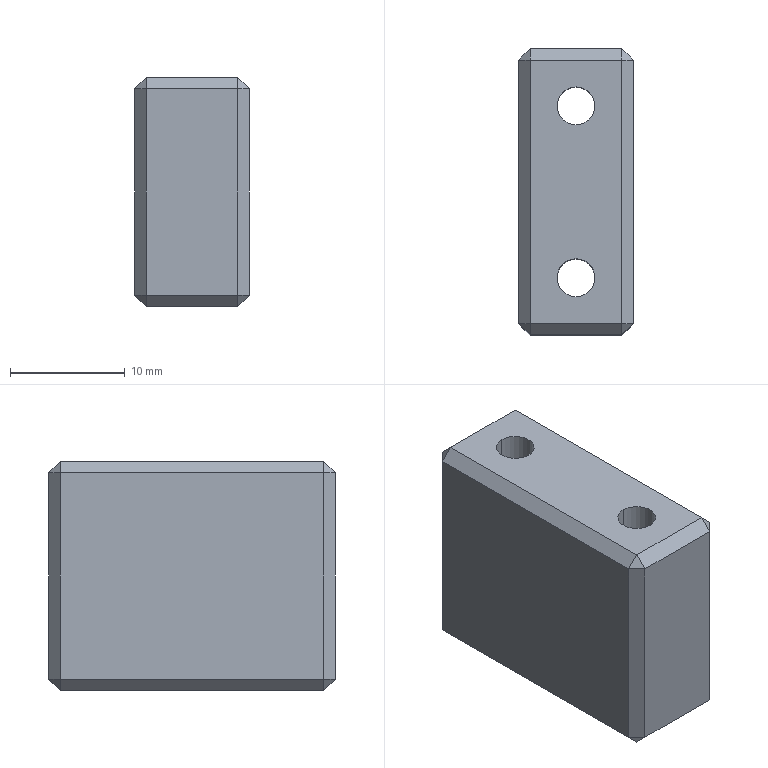Component | SolidWorks | SL010-RightStreamline-1-1_SL010-BeltMotorAssembly-1-1_SL010-LXFB-0102008-1-2 | 1 solid | 30 faces | box 10 x 25 x 20 mm | volume 4553 mm3 | plane 26 | cylinder 4 | commonest cylinder face diameters 3.3 x4 | material Aluminum-6061
build123d program:
from build123d import *

# Parameters (mm, degrees)
SKETCH1_W           = 10
SKETCH1_H           = 25
BOSS_EXTRUDE1_DEPTH = 10
M4_TAPPED_HOLE1_D   = 3.3
CHAMFER1_SIZE       = 1


with BuildPart() as part:
    # Sketch1 → Boss-Extrude1 (new, symmetric)
    with BuildSketch(Plane(origin=(0, 0, 0), x_dir=(1, 0, 0), z_dir=(0, 1, 0))):
        Rectangle(SKETCH1_W, SKETCH1_H)
    extrude(amount=BOSS_EXTRUDE1_DEPTH, both=True)

    # M4 Tapped Hole1 (through all)
    with Locations(Plane(origin=(0, 10, 0), x_dir=(1, 0, 0), z_dir=(0, 1, 0))):
        with Locations((0, -7.5), (0, 7.5)):
            Hole(M4_TAPPED_HOLE1_D / 2)

    # Chamfer1
    chamfer1_edges = [part.edges().sort_by_distance(p)[0] for p in [
        (5, 10, 0),
        (0, 10, -12.5),
        (-5, 10, 0),
        (0, -10, -12.5),
        (5, -10, 0),
        (0, -10, 12.5),
        (-5, -10, 0),
        (0, 10, 12.5),
        (-5, 0, -12.5),
        (5, 0, -12.5),
        (5, 0, 12.5),
        (-5, 0, 12.5),
    ]]
    chamfer(chamfer1_edges, length=CHAMFER1_SIZE)


solid = part.part

# Placed as in the assembly
solid = solid.moved(Location((-547.5, -215.404, -306.035), (90, 0, 0)))
STEP:
#1=COLOUR_RGB('',0.7922,0.8196,0.9333);
#2=FILL_AREA_STYLE_COLOUR('',#1);
#3=FILL_AREA_STYLE('',(#2));
#4=SURFACE_STYLE_FILL_AREA(#3);
#5=SURFACE_SIDE_STYLE('',(#4));
#6=SURFACE_STYLE_USAGE(.BOTH.,#5);
#7=PRESENTATION_STYLE_ASSIGNMENT((#6));
#8=CARTESIAN_POINT('',(-21.555,-8.25,-12.442));
#9=VERTEX_POINT('',#8);
#10=CARTESIAN_POINT('',(-21.555,-8.12,-12.442));
#11=VERTEX_POINT('',#10);
#12=CARTESIAN_POINT('',(-21.555,-8.185,-12.442));
#13=DIRECTION('',(0.,-0.,1.));
#14=DIRECTION('',(0.,1.,0.));
#15=AXIS2_PLACEMENT_3D('',#12,#13,#14);
#16=CIRCLE('',#15,0.06496);
#17=EDGE_CURVE('',#9,#11,#16,.T.);
#18=ORIENTED_EDGE('',*,*,#17,.F.);
#19=CARTESIAN_POINT('',(-21.555,-8.25,-11.655));
#20=VERTEX_POINT('',#19);
#21=CARTESIAN_POINT('',(-21.555,-8.25,-11.655));
#22=DIRECTION('',(0.,-0.,1.));
#23=VECTOR('',#22,39.37);
#24=LINE('',#21,#23);
#25=EDGE_CURVE('',#9,#20,#24,.T.);
#26=ORIENTED_EDGE('',*,*,#25,.T.);
#27=CARTESIAN_POINT('',(-21.555,-8.12,-11.655));
#28=VERTEX_POINT('',#27);
#29=CARTESIAN_POINT('',(-21.555,-8.185,-11.655));
#30=DIRECTION('',(0.,-0.,1.));
#31=DIRECTION('',(0.,1.,0.));
#32=AXIS2_PLACEMENT_3D('',#29,#30,#31);
#33=CIRCLE('',#32,0.06496);
#34=EDGE_CURVE('',#20,#28,#33,.T.);
#35=ORIENTED_EDGE('',*,*,#34,.T.);
#36=CARTESIAN_POINT('',(-21.555,-8.12,-11.655));
#37=DIRECTION('',(0.,-0.,1.));
#38=VECTOR('',#37,39.37);
#39=LINE('',#36,#38);
#40=EDGE_CURVE('',#11,#28,#39,.T.);
#41=ORIENTED_EDGE('',*,*,#40,.F.);
#42=EDGE_LOOP('',(#18,#26,#35,#41));
#43=FACE_OUTER_BOUND('',#42,.T.);
#44=CARTESIAN_POINT('',(-21.555,-8.185,-11.655));
#45=DIRECTION('',(0.,-0.,1.));
#46=DIRECTION('',(0.,1.,0.));
#47=AXIS2_PLACEMENT_3D('',#44,#45,#46);
#48=CYLINDRICAL_SURFACE('',#47,0.06496);
#49=ADVANCED_FACE('',(#43),#48,.F.);
#50=CARTESIAN_POINT('',(-21.555,-8.841,-12.442));
#51=VERTEX_POINT('',#50);
#52=CARTESIAN_POINT('',(-21.555,-8.711,-12.442));
#53=VERTEX_POINT('',#52);
#54=CARTESIAN_POINT('',(-21.555,-8.776,-12.442));
#55=DIRECTION('',(0.,-0.,1.));
#56=DIRECTION('',(0.,1.,0.));
#57=AXIS2_PLACEMENT_3D('',#54,#55,#56);
#58=CIRCLE('',#57,0.06496);
#59=EDGE_CURVE('',#51,#53,#58,.T.);
#60=ORIENTED_EDGE('',*,*,#59,.F.);
#61=CARTESIAN_POINT('',(-21.555,-8.841,-11.655));
#62=VERTEX_POINT('',#61);
#63=CARTESIAN_POINT('',(-21.555,-8.841,-11.655));
#64=DIRECTION('',(0.,-0.,1.));
#65=VECTOR('',#64,39.37);
#66=LINE('',#63,#65);
#67=EDGE_CURVE('',#51,#62,#66,.T.);
#68=ORIENTED_EDGE('',*,*,#67,.T.);
#69=CARTESIAN_POINT('',(-21.555,-8.711,-11.655));
#70=VERTEX_POINT('',#69);
#71=CARTESIAN_POINT('',(-21.555,-8.776,-11.655));
#72=DIRECTION('',(0.,-0.,1.));
#73=DIRECTION('',(0.,1.,0.));
#74=AXIS2_PLACEMENT_3D('',#71,#72,#73);
#75=CIRCLE('',#74,0.06496);
#76=EDGE_CURVE('',#62,#70,#75,.T.);
#77=ORIENTED_EDGE('',*,*,#76,.T.);
#78=CARTESIAN_POINT('',(-21.555,-8.711,-11.655));
#79=DIRECTION('',(0.,-0.,1.));
#80=VECTOR('',#79,39.37);
#81=LINE('',#78,#80);
#82=EDGE_CURVE('',#53,#70,#81,.T.);
#83=ORIENTED_EDGE('',*,*,#82,.F.);
#84=EDGE_LOOP('',(#60,#68,#77,#83));
#85=FACE_OUTER_BOUND('',#84,.T.);
#86=CARTESIAN_POINT('',(-21.555,-8.776,-11.655));
#87=DIRECTION('',(0.,-0.,1.));
#88=DIRECTION('',(0.,1.,0.));
#89=AXIS2_PLACEMENT_3D('',#86,#87,#88);
#90=CYLINDRICAL_SURFACE('',#89,0.06496);
#91=ADVANCED_FACE('',(#85),#90,.F.);
#92=CARTESIAN_POINT('',(-21.358,-8.028,-11.694));
#93=VERTEX_POINT('',#92);
#94=CARTESIAN_POINT('',(-21.358,-8.933,-11.694));
#95=VERTEX_POINT('',#94);
#96=CARTESIAN_POINT('',(-21.358,-8.973,-11.694));
#97=DIRECTION('',(-0.,-1.,-0.));
#98=VECTOR('',#97,39.37);
#99=LINE('',#96,#98);
#100=EDGE_CURVE('',#93,#95,#99,.T.);
#101=ORIENTED_EDGE('',*,*,#100,.T.);
#102=CARTESIAN_POINT('',(-21.358,-8.933,-12.403));
#103=VERTEX_POINT('',#102);
#104=CARTESIAN_POINT('',(-21.358,-8.933,-11.655));
#105=DIRECTION('',(0.,0.,-1.));
#106=VECTOR('',#105,39.37);
#107=LINE('',#104,#106);
#108=EDGE_CURVE('',#95,#103,#107,.T.);
#109=ORIENTED_EDGE('',*,*,#108,.T.);
#110=CARTESIAN_POINT('',(-21.358,-8.028,-12.403));
#111=VERTEX_POINT('',#110);
#112=CARTESIAN_POINT('',(-21.358,-7.988,-12.403));
#113=DIRECTION('',(0.,1.,0.));
#114=VECTOR('',#113,39.37);
#115=LINE('',#112,#114);
#116=EDGE_CURVE('',#103,#111,#115,.T.);
#117=ORIENTED_EDGE('',*,*,#116,.T.);
#118=CARTESIAN_POINT('',(-21.358,-8.028,-11.655));
#119=DIRECTION('',(0.,-0.,1.));
#120=VECTOR('',#119,39.37);
#121=LINE('',#118,#120);
#122=EDGE_CURVE('',#111,#93,#121,.T.);
#123=ORIENTED_EDGE('',*,*,#122,.T.);
#124=EDGE_LOOP('',(#101,#109,#117,#123));
#125=FACE_OUTER_BOUND('',#124,.T.);
#126=CARTESIAN_POINT('',(-21.358,-7.988,-11.655));
#127=DIRECTION('',(-1.,0.,-0.));
#128=DIRECTION('',(-0.,-1.,-0.));
#129=AXIS2_PLACEMENT_3D('',#126,#127,#128);
#130=PLANE('',#129);
#131=ADVANCED_FACE('',(#125),#130,.F.);
#132=CARTESIAN_POINT('',(-21.398,-7.988,-12.403));
#133=VERTEX_POINT('',#132);
#134=CARTESIAN_POINT('',(-21.713,-7.988,-12.403));
#135=VERTEX_POINT('',#134);
#136=CARTESIAN_POINT('',(-21.752,-7.988,-12.403));
#137=DIRECTION('',(-1.,-0.,-0.));
#138=VECTOR('',#137,39.37);
#139=LINE('',#136,#138);
#140=EDGE_CURVE('',#133,#135,#139,.T.);
#141=ORIENTED_EDGE('',*,*,#140,.T.);
#142=CARTESIAN_POINT('',(-21.713,-7.988,-11.694));
#143=VERTEX_POINT('',#142);
#144=CARTESIAN_POINT('',(-21.713,-7.988,-11.655));
#145=DIRECTION('',(0.,-0.,1.));
#146=VECTOR('',#145,39.37);
#147=LINE('',#144,#146);
#148=EDGE_CURVE('',#135,#143,#147,.T.);
#149=ORIENTED_EDGE('',*,*,#148,.T.);
#150=CARTESIAN_POINT('',(-21.398,-7.988,-11.694));
#151=VERTEX_POINT('',#150);
#152=CARTESIAN_POINT('',(-21.358,-7.988,-11.694));
#153=DIRECTION('',(1.,0.,0.));
#154=VECTOR('',#153,39.37);
#155=LINE('',#152,#154);
#156=EDGE_CURVE('',#143,#151,#155,.T.);
#157=ORIENTED_EDGE('',*,*,#156,.T.);
#158=CARTESIAN_POINT('',(-21.398,-7.988,-11.655));
#159=DIRECTION('',(0.,0.,-1.));
#160=VECTOR('',#159,39.37);
#161=LINE('',#158,#160);
#162=EDGE_CURVE('',#151,#133,#161,.T.);
#163=ORIENTED_EDGE('',*,*,#162,.T.);
#164=EDGE_LOOP('',(#141,#149,#157,#163));
#165=FACE_OUTER_BOUND('',#164,.T.);
#166=CARTESIAN_POINT('',(-21.752,-7.988,-11.655));
#167=DIRECTION('',(0.,-1.,-0.));
#168=DIRECTION('',(1.,0.,0.));
#169=AXIS2_PLACEMENT_3D('',#166,#167,#168);
#170=PLANE('',#169);
#171=ADVANCED_FACE('',(#165),#170,.F.);
#172=CARTESIAN_POINT('',(-21.752,-8.933,-11.694));
#173=VERTEX_POINT('',#172);
#174=CARTESIAN_POINT('',(-21.752,-8.028,-11.694));
#175=VERTEX_POINT('',#174);
#176=CARTESIAN_POINT('',(-21.752,-7.988,-11.694));
#177=DIRECTION('',(0.,1.,0.));
#178=VECTOR('',#177,39.37);
#179=LINE('',#176,#178);
#180=EDGE_CURVE('',#173,#175,#179,.T.);
#181=ORIENTED_EDGE('',*,*,#180,.T.);
#182=CARTESIAN_POINT('',(-21.752,-8.028,-12.403));
#183=VERTEX_POINT('',#182);
#184=CARTESIAN_POINT('',(-21.752,-8.028,-11.655));
#185=DIRECTION('',(0.,0.,-1.));
#186=VECTOR('',#185,39.37);
#187=LINE('',#184,#186);
#188=EDGE_CURVE('',#175,#183,#187,.T.);
#189=ORIENTED_EDGE('',*,*,#188,.T.);
#190=CARTESIAN_POINT('',(-21.752,-8.933,-12.403));
#191=VERTEX_POINT('',#190);
#192=CARTESIAN_POINT('',(-21.752,-7.988,-12.403));
#193=DIRECTION('',(-0.,-1.,-0.));
#194=VECTOR('',#193,39.37);
#195=LINE('',#192,#194);
#196=EDGE_CURVE('',#183,#191,#195,.T.);
#197=ORIENTED_EDGE('',*,*,#196,.T.);
#198=CARTESIAN_POINT('',(-21.752,-8.933,-11.655));
#199=DIRECTION('',(0.,-0.,1.));
#200=VECTOR('',#199,39.37);
#201=LINE('',#198,#200);
#202=EDGE_CURVE('',#191,#173,#201,.T.);
#203=ORIENTED_EDGE('',*,*,#202,.T.);
#204=EDGE_LOOP('',(#181,#189,#197,#203));
#205=FACE_OUTER_BOUND('',#204,.T.);
#206=CARTESIAN_POINT('',(-21.752,-7.988,-11.655));
#207=DIRECTION('',(1.,-0.,0.));
#208=DIRECTION('',(0.,1.,0.));
#209=AXIS2_PLACEMENT_3D('',#206,#207,#208);
#210=PLANE('',#209);
#211=ADVANCED_FACE('',(#205),#210,.F.);
#212=CARTESIAN_POINT('',(-21.398,-8.973,-12.403));
#213=VERTEX_POINT('',#212);
#214=CARTESIAN_POINT('',(-21.398,-8.973,-11.694));
#215=VERTEX_POINT('',#214);
#216=CARTESIAN_POINT('',(-21.398,-8.973,-11.655));
#217=DIRECTION('',(0.,-0.,1.));
#218=VECTOR('',#217,39.37);
#219=LINE('',#216,#218);
#220=EDGE_CURVE('',#213,#215,#219,.T.);
#221=ORIENTED_EDGE('',*,*,#220,.T.);
#222=CARTESIAN_POINT('',(-21.713,-8.973,-11.694));
#223=VERTEX_POINT('',#222);
#224=CARTESIAN_POINT('',(-21.752,-8.973,-11.694));
#225=DIRECTION('',(-1.,0.,-0.));
#226=VECTOR('',#225,39.37);
#227=LINE('',#224,#226);
#228=EDGE_CURVE('',#215,#223,#227,.T.);
#229=ORIENTED_EDGE('',*,*,#228,.T.);
#230=CARTESIAN_POINT('',(-21.713,-8.973,-12.403));
#231=VERTEX_POINT('',#230);
#232=CARTESIAN_POINT('',(-21.713,-8.973,-11.655));
#233=DIRECTION('',(0.,0.,-1.));
#234=VECTOR('',#233,39.37);
#235=LINE('',#232,#234);
#236=EDGE_CURVE('',#223,#231,#235,.T.);
#237=ORIENTED_EDGE('',*,*,#236,.T.);
#238=CARTESIAN_POINT('',(-21.752,-8.973,-12.403));
#239=DIRECTION('',(1.,-0.,0.));
#240=VECTOR('',#239,39.37);
#241=LINE('',#238,#240);
#242=EDGE_CURVE('',#231,#213,#241,.T.);
#243=ORIENTED_EDGE('',*,*,#242,.T.);
#244=EDGE_LOOP('',(#221,#229,#237,#243));
#245=FACE_OUTER_BOUND('',#244,.T.);
#246=CARTESIAN_POINT('',(-21.752,-8.973,-11.655));
#247=DIRECTION('',(0.,1.,0.));
#248=DIRECTION('',(-1.,0.,-0.));
#249=AXIS2_PLACEMENT_3D('',#246,#247,#248);
#250=PLANE('',#249);
#251=ADVANCED_FACE('',(#245),#250,.F.);
#252=CARTESIAN_POINT('',(-21.398,-8.028,-11.655));
#253=VERTEX_POINT('',#252);
#254=CARTESIAN_POINT('',(-21.713,-8.028,-11.655));
#255=VERTEX_POINT('',#254);
#256=CARTESIAN_POINT('',(-21.752,-8.028,-11.655));
#257=DIRECTION('',(-1.,-0.,-0.));
#258=VECTOR('',#257,39.37);
#259=LINE('',#256,#258);
#260=EDGE_CURVE('',#253,#255,#259,.T.);
#261=ORIENTED_EDGE('',*,*,#260,.T.);
#262=CARTESIAN_POINT('',(-21.713,-8.933,-11.655));
#263=VERTEX_POINT('',#262);
#264=CARTESIAN_POINT('',(-21.713,-8.973,-11.655));
#265=DIRECTION('',(-0.,-1.,-0.));
#266=VECTOR('',#265,39.37);
#267=LINE('',#264,#266);
#268=EDGE_CURVE('',#255,#263,#267,.T.);
#269=ORIENTED_EDGE('',*,*,#268,.T.);
#270=CARTESIAN_POINT('',(-21.398,-8.933,-11.655));
#271=VERTEX_POINT('',#270);
#272=CARTESIAN_POINT('',(-21.358,-8.933,-11.655));
#273=DIRECTION('',(1.,-0.,0.));
#274=VECTOR('',#273,39.37);
#275=LINE('',#272,#274);
#276=EDGE_CURVE('',#263,#271,#275,.T.);
#277=ORIENTED_EDGE('',*,*,#276,.T.);
#278=CARTESIAN_POINT('',(-21.398,-7.988,-11.655));
#279=DIRECTION('',(0.,1.,0.));
#280=VECTOR('',#279,39.37);
#281=LINE('',#278,#280);
#282=EDGE_CURVE('',#271,#253,#281,.T.);
#283=ORIENTED_EDGE('',*,*,#282,.T.);
#284=EDGE_LOOP('',(#261,#269,#277,#283));
#285=FACE_OUTER_BOUND('',#284,.T.);
#286=CARTESIAN_POINT('',(-21.555,-8.185,-11.655));
#287=DIRECTION('',(0.,-0.,1.));
#288=DIRECTION('',(0.,1.,0.));
#289=AXIS2_PLACEMENT_3D('',#286,#287,#288);
#290=CIRCLE('',#289,0.06496);
#291=EDGE_CURVE('',#28,#20,#290,.T.);
#292=ORIENTED_EDGE('',*,*,#291,.F.);
#293=ORIENTED_EDGE('',*,*,#34,.F.);
#294=EDGE_LOOP('',(#292,#293));
#295=FACE_BOUND('',#294,.T.);
#296=CARTESIAN_POINT('',(-21.555,-8.776,-11.655));
#297=DIRECTION('',(0.,-0.,1.));
#298=DIRECTION('',(0.,1.,0.));
#299=AXIS2_PLACEMENT_3D('',#296,#297,#298);
#300=CIRCLE('',#299,0.06496);
#301=EDGE_CURVE('',#70,#62,#300,.T.);
#302=ORIENTED_EDGE('',*,*,#301,.F.);
#303=ORIENTED_EDGE('',*,*,#76,.F.);
#304=EDGE_LOOP('',(#302,#303));
#305=FACE_BOUND('',#304,.T.);
#306=CARTESIAN_POINT('',(-21.555,-8.48,-11.655));
#307=DIRECTION('',(-0.,-0.,1.));
#308=DIRECTION('',(0.,1.,0.));
#309=AXIS2_PLACEMENT_3D('',#306,#307,#308);
#310=PLANE('',#309);
#311=ADVANCED_FACE('',(#285,#295,#305),#310,.T.);
#312=CARTESIAN_POINT('',(-21.713,-8.933,-12.442));
#313=VERTEX_POINT('',#312);
#314=CARTESIAN_POINT('',(-21.713,-8.028,-12.442));
#315=VERTEX_POINT('',#314);
#316=CARTESIAN_POINT('',(-21.713,-8.48,-12.442));
#317=DIRECTION('',(0.,1.,0.));
#318=VECTOR('',#317,39.37);
#319=LINE('',#316,#318);
#320=EDGE_CURVE('',#313,#315,#319,.T.);
#321=ORIENTED_EDGE('',*,*,#320,.T.);
#322=CARTESIAN_POINT('',(-21.398,-8.028,-12.442));
#323=VERTEX_POINT('',#322);
#324=CARTESIAN_POINT('',(-21.555,-8.028,-12.442));
#325=DIRECTION('',(1.,0.,0.));
#326=VECTOR('',#325,39.37);
#327=LINE('',#324,#326);
#328=EDGE_CURVE('',#315,#323,#327,.T.);
#329=ORIENTED_EDGE('',*,*,#328,.T.);
#330=CARTESIAN_POINT('',(-21.398,-8.933,-12.442));
#331=VERTEX_POINT('',#330);
#332=CARTESIAN_POINT('',(-21.398,-8.48,-12.442));
#333=DIRECTION('',(-0.,-1.,-0.));
#334=VECTOR('',#333,39.37);
#335=LINE('',#332,#334);
#336=EDGE_CURVE('',#323,#331,#335,.T.);
#337=ORIENTED_EDGE('',*,*,#336,.T.);
#338=CARTESIAN_POINT('',(-21.555,-8.933,-12.442));
#339=DIRECTION('',(-1.,0.,-0.));
#340=VECTOR('',#339,39.37);
#341=LINE('',#338,#340);
#342=EDGE_CURVE('',#331,#313,#341,.T.);
#343=ORIENTED_EDGE('',*,*,#342,.T.);
#344=EDGE_LOOP('',(#321,#329,#337,#343));
#345=FACE_OUTER_BOUND('',#344,.T.);
#346=CARTESIAN_POINT('',(-21.555,-8.185,-12.442));
#347=DIRECTION('',(0.,-0.,1.));
#348=DIRECTION('',(0.,1.,0.));
#349=AXIS2_PLACEMENT_3D('',#346,#347,#348);
#350=CIRCLE('',#349,0.06496);
#351=EDGE_CURVE('',#11,#9,#350,.T.);
#352=ORIENTED_EDGE('',*,*,#351,.T.);
#353=ORIENTED_EDGE('',*,*,#17,.T.);
#354=EDGE_LOOP('',(#352,#353));
#355=FACE_BOUND('',#354,.T.);
#356=CARTESIAN_POINT('',(-21.555,-8.776,-12.442));
#357=DIRECTION('',(0.,-0.,1.));
#358=DIRECTION('',(0.,1.,0.));
#359=AXIS2_PLACEMENT_3D('',#356,#357,#358);
#360=CIRCLE('',#359,0.06496);
#361=EDGE_CURVE('',#53,#51,#360,.T.);
#362=ORIENTED_EDGE('',*,*,#361,.T.);
#363=ORIENTED_EDGE('',*,*,#59,.T.);
#364=EDGE_LOOP('',(#362,#363));
#365=FACE_BOUND('',#364,.T.);
#366=CARTESIAN_POINT('',(-21.555,-8.48,-12.442));
#367=DIRECTION('',(-0.,-0.,1.));
#368=DIRECTION('',(0.,1.,0.));
#369=AXIS2_PLACEMENT_3D('',#366,#367,#368);
#370=PLANE('',#369);
#371=ADVANCED_FACE('',(#345,#355,#365),#370,.F.);
#372=ORIENTED_EDGE('',*,*,#67,.F.);
#373=ORIENTED_EDGE('',*,*,#361,.F.);
#374=ORIENTED_EDGE('',*,*,#82,.T.);
#375=ORIENTED_EDGE('',*,*,#301,.T.);
#376=EDGE_LOOP('',(#372,#373,#374,#375));
#377=FACE_OUTER_BOUND('',#376,.T.);
#378=CARTESIAN_POINT('',(-21.555,-8.776,-11.655));
#379=DIRECTION('',(0.,-0.,1.));
#380=DIRECTION('',(0.,1.,0.));
#381=AXIS2_PLACEMENT_3D('',#378,#379,#380);
#382=CYLINDRICAL_SURFACE('',#381,0.06496);
#383=ADVANCED_FACE('',(#377),#382,.F.);
#384=ORIENTED_EDGE('',*,*,#25,.F.);
#385=ORIENTED_EDGE('',*,*,#351,.F.);
#386=ORIENTED_EDGE('',*,*,#40,.T.);
#387=ORIENTED_EDGE('',*,*,#291,.T.);
#388=EDGE_LOOP('',(#384,#385,#386,#387));
#389=FACE_OUTER_BOUND('',#388,.T.);
#390=CARTESIAN_POINT('',(-21.555,-8.185,-11.655));
#391=DIRECTION('',(0.,-0.,1.));
#392=DIRECTION('',(0.,1.,0.));
#393=AXIS2_PLACEMENT_3D('',#390,#391,#392);
#394=CYLINDRICAL_SURFACE('',#393,0.06496);
#395=ADVANCED_FACE('',(#389),#394,.F.);
#396=CARTESIAN_POINT('',(-21.398,-8.973,-12.403));
#397=DIRECTION('',(0.,0.7071,-0.7071));
#398=VECTOR('',#397,39.37);
#399=LINE('',#396,#398);
#400=EDGE_CURVE('',#213,#331,#399,.T.);
#401=ORIENTED_EDGE('',*,*,#400,.F.);
#402=ORIENTED_EDGE('',*,*,#242,.F.);
#403=CARTESIAN_POINT('',(-21.713,-8.973,-12.403));
#404=DIRECTION('',(-0.,-0.7071,0.7071));
#405=VECTOR('',#404,39.37);
#406=LINE('',#403,#405);
#407=EDGE_CURVE('',#313,#231,#406,.T.);
#408=ORIENTED_EDGE('',*,*,#407,.F.);
#409=ORIENTED_EDGE('',*,*,#342,.F.);
#410=EDGE_LOOP('',(#401,#402,#408,#409));
#411=FACE_OUTER_BOUND('',#410,.T.);
#412=CARTESIAN_POINT('',(-21.752,-8.973,-12.403));
#413=DIRECTION('',(0.,0.7071,0.7071));
#414=DIRECTION('',(1.,-0.,0.));
#415=AXIS2_PLACEMENT_3D('',#412,#413,#414);
#416=PLANE('',#415);
#417=ADVANCED_FACE('',(#411),#416,.F.);
#418=CARTESIAN_POINT('',(-21.398,-8.973,-12.403));
#419=DIRECTION('',(0.7071,0.7071,0.));
#420=VECTOR('',#419,39.37);
#421=LINE('',#418,#420);
#422=EDGE_CURVE('',#213,#103,#421,.T.);
#423=ORIENTED_EDGE('',*,*,#422,.F.);
#424=ORIENTED_EDGE('',*,*,#400,.T.);
#425=CARTESIAN_POINT('',(-21.378,-8.933,-12.423));
#426=DIRECTION('',(-0.7071,0.,-0.7071));
#427=VECTOR('',#426,39.37);
#428=LINE('',#425,#427);
#429=EDGE_CURVE('',#103,#331,#428,.T.);
#430=ORIENTED_EDGE('',*,*,#429,.F.);
#431=EDGE_LOOP('',(#423,#424,#430));
#432=FACE_OUTER_BOUND('',#431,.T.);
#433=CARTESIAN_POINT('',(-21.398,-8.973,-12.403));
#434=DIRECTION('',(0.5774,-0.5774,-0.5774));
#435=DIRECTION('',(-0.,-0.7071,0.7071));
#436=AXIS2_PLACEMENT_3D('',#433,#434,#435);
#437=PLANE('',#436);
#438=ADVANCED_FACE('',(#432),#437,.T.);
#439=CARTESIAN_POINT('',(-21.732,-8.933,-12.423));
#440=DIRECTION('',(-0.7071,0.,0.7071));
#441=VECTOR('',#440,39.37);
#442=LINE('',#439,#441);
#443=EDGE_CURVE('',#313,#191,#442,.T.);
#444=ORIENTED_EDGE('',*,*,#443,.F.);
#445=ORIENTED_EDGE('',*,*,#407,.T.);
#446=CARTESIAN_POINT('',(-21.713,-8.973,-12.403));
#447=DIRECTION('',(0.7071,-0.7071,-0.));
#448=VECTOR('',#447,39.37);
#449=LINE('',#446,#448);
#450=EDGE_CURVE('',#191,#231,#449,.T.);
#451=ORIENTED_EDGE('',*,*,#450,.F.);
#452=EDGE_LOOP('',(#444,#445,#451));
#453=FACE_OUTER_BOUND('',#452,.T.);
#454=CARTESIAN_POINT('',(-21.713,-8.973,-12.403));
#455=DIRECTION('',(-0.5774,-0.5774,-0.5774));
#456=DIRECTION('',(0.7071,-0.7071,-0.));
#457=AXIS2_PLACEMENT_3D('',#454,#455,#456);
#458=PLANE('',#457);
#459=ADVANCED_FACE('',(#453),#458,.T.);
#460=ORIENTED_EDGE('',*,*,#429,.T.);
#461=ORIENTED_EDGE('',*,*,#336,.F.);
#462=CARTESIAN_POINT('',(-21.398,-8.028,-12.442));
#463=DIRECTION('',(-0.7071,-0.,-0.7071));
#464=VECTOR('',#463,39.37);
#465=LINE('',#462,#464);
#466=EDGE_CURVE('',#111,#323,#465,.T.);
#467=ORIENTED_EDGE('',*,*,#466,.F.);
#468=ORIENTED_EDGE('',*,*,#116,.F.);
#469=EDGE_LOOP('',(#460,#461,#467,#468));
#470=FACE_OUTER_BOUND('',#469,.T.);
#471=CARTESIAN_POINT('',(-21.358,-7.988,-12.403));
#472=DIRECTION('',(-0.7071,0.,0.7071));
#473=DIRECTION('',(0.,1.,0.));
#474=AXIS2_PLACEMENT_3D('',#471,#472,#473);
#475=PLANE('',#474);
#476=ADVANCED_FACE('',(#470),#475,.F.);
#477=ORIENTED_EDGE('',*,*,#422,.T.);
#478=ORIENTED_EDGE('',*,*,#108,.F.);
#479=CARTESIAN_POINT('',(-21.378,-8.953,-11.694));
#480=DIRECTION('',(0.7071,0.7071,0.));
#481=VECTOR('',#480,39.37);
#482=LINE('',#479,#481);
#483=EDGE_CURVE('',#215,#95,#482,.T.);
#484=ORIENTED_EDGE('',*,*,#483,.F.);
#485=ORIENTED_EDGE('',*,*,#220,.F.);
#486=EDGE_LOOP('',(#477,#478,#484,#485));
#487=FACE_OUTER_BOUND('',#486,.T.);
#488=CARTESIAN_POINT('',(-21.358,-8.933,-11.655));
#489=DIRECTION('',(-0.7071,0.7071,0.));
#490=DIRECTION('',(0.,0.,-1.));
#491=AXIS2_PLACEMENT_3D('',#488,#489,#490);
#492=PLANE('',#491);
#493=ADVANCED_FACE('',(#487),#492,.F.);
#494=CARTESIAN_POINT('',(-21.713,-8.973,-11.694));
#495=DIRECTION('',(0.,0.7071,0.7071));
#496=VECTOR('',#495,39.37);
#497=LINE('',#494,#496);
#498=EDGE_CURVE('',#223,#263,#497,.T.);
#499=ORIENTED_EDGE('',*,*,#498,.F.);
#500=ORIENTED_EDGE('',*,*,#228,.F.);
#501=CARTESIAN_POINT('',(-21.398,-8.933,-11.655));
#502=DIRECTION('',(-0.,-0.7071,-0.7071));
#503=VECTOR('',#502,39.37);
#504=LINE('',#501,#503);
#505=EDGE_CURVE('',#271,#215,#504,.T.);
#506=ORIENTED_EDGE('',*,*,#505,.F.);
#507=ORIENTED_EDGE('',*,*,#276,.F.);
#508=EDGE_LOOP('',(#499,#500,#506,#507));
#509=FACE_OUTER_BOUND('',#508,.T.);
#510=CARTESIAN_POINT('',(-21.555,-8.933,-11.655));
#511=DIRECTION('',(-0.,-0.7071,0.7071));
#512=DIRECTION('',(-1.,0.,-0.));
#513=AXIS2_PLACEMENT_3D('',#510,#511,#512);
#514=PLANE('',#513);
#515=ADVANCED_FACE('',(#509),#514,.T.);
#516=ORIENTED_EDGE('',*,*,#450,.T.);
#517=ORIENTED_EDGE('',*,*,#236,.F.);
#518=CARTESIAN_POINT('',(-21.713,-8.973,-11.694));
#519=DIRECTION('',(0.7071,-0.7071,-0.));
#520=VECTOR('',#519,39.37);
#521=LINE('',#518,#520);
#522=EDGE_CURVE('',#173,#223,#521,.T.);
#523=ORIENTED_EDGE('',*,*,#522,.F.);
#524=ORIENTED_EDGE('',*,*,#202,.F.);
#525=EDGE_LOOP('',(#516,#517,#523,#524));
#526=FACE_OUTER_BOUND('',#525,.T.);
#527=CARTESIAN_POINT('',(-21.713,-8.973,-11.655));
#528=DIRECTION('',(0.7071,0.7071,0.));
#529=DIRECTION('',(0.,0.,-1.));
#530=AXIS2_PLACEMENT_3D('',#527,#528,#529);
#531=PLANE('',#530);
#532=ADVANCED_FACE('',(#526),#531,.F.);
#533=ORIENTED_EDGE('',*,*,#443,.T.);
#534=ORIENTED_EDGE('',*,*,#196,.F.);
#535=CARTESIAN_POINT('',(-21.732,-8.028,-12.423));
#536=DIRECTION('',(-0.7071,0.,0.7071));
#537=VECTOR('',#536,39.37);
#538=LINE('',#535,#537);
#539=EDGE_CURVE('',#315,#183,#538,.T.);
#540=ORIENTED_EDGE('',*,*,#539,.F.);
#541=ORIENTED_EDGE('',*,*,#320,.F.);
#542=EDGE_LOOP('',(#533,#534,#540,#541));
#543=FACE_OUTER_BOUND('',#542,.T.);
#544=CARTESIAN_POINT('',(-21.752,-7.988,-12.403));
#545=DIRECTION('',(0.7071,-0.,0.7071));
#546=DIRECTION('',(-0.,-1.,-0.));
#547=AXIS2_PLACEMENT_3D('',#544,#545,#546);
#548=PLANE('',#547);
#549=ADVANCED_FACE('',(#543),#548,.F.);
#550=CARTESIAN_POINT('',(-21.398,-8.028,-12.442));
#551=DIRECTION('',(-0.,0.7071,0.7071));
#552=VECTOR('',#551,39.37);
#553=LINE('',#550,#552);
#554=EDGE_CURVE('',#323,#133,#553,.T.);
#555=ORIENTED_EDGE('',*,*,#554,.F.);
#556=ORIENTED_EDGE('',*,*,#328,.F.);
#557=CARTESIAN_POINT('',(-21.713,-7.988,-12.403));
#558=DIRECTION('',(0.,-0.7071,-0.7071));
#559=VECTOR('',#558,39.37);
#560=LINE('',#557,#559);
#561=EDGE_CURVE('',#135,#315,#560,.T.);
#562=ORIENTED_EDGE('',*,*,#561,.F.);
#563=ORIENTED_EDGE('',*,*,#140,.F.);
#564=EDGE_LOOP('',(#555,#556,#562,#563));
#565=FACE_OUTER_BOUND('',#564,.T.);
#566=CARTESIAN_POINT('',(-21.752,-7.988,-12.403));
#567=DIRECTION('',(0.,-0.7071,0.7071));
#568=DIRECTION('',(-1.,-0.,-0.));
#569=AXIS2_PLACEMENT_3D('',#566,#567,#568);
#570=PLANE('',#569);
#571=ADVANCED_FACE('',(#565),#570,.F.);
#572=ORIENTED_EDGE('',*,*,#466,.T.);
#573=ORIENTED_EDGE('',*,*,#554,.T.);
#574=CARTESIAN_POINT('',(-21.378,-8.008,-12.403));
#575=DIRECTION('',(-0.7071,0.7071,0.));
#576=VECTOR('',#575,39.37);
#577=LINE('',#574,#576);
#578=EDGE_CURVE('',#111,#133,#577,.T.);
#579=ORIENTED_EDGE('',*,*,#578,.F.);
#580=EDGE_LOOP('',(#572,#573,#579));
#581=FACE_OUTER_BOUND('',#580,.T.);
#582=CARTESIAN_POINT('',(-21.398,-8.028,-12.442));
#583=DIRECTION('',(0.5774,0.5774,-0.5774));
#584=DIRECTION('',(-0.,-0.7071,-0.7071));
#585=AXIS2_PLACEMENT_3D('',#582,#583,#584);
#586=PLANE('',#585);
#587=ADVANCED_FACE('',(#581),#586,.T.);
#588=ORIENTED_EDGE('',*,*,#505,.T.);
#589=ORIENTED_EDGE('',*,*,#483,.T.);
#590=CARTESIAN_POINT('',(-21.398,-8.933,-11.655));
#591=DIRECTION('',(0.7071,-0.,-0.7071));
#592=VECTOR('',#591,39.37);
#593=LINE('',#590,#592);
#594=EDGE_CURVE('',#271,#95,#593,.T.);
#595=ORIENTED_EDGE('',*,*,#594,.F.);
#596=EDGE_LOOP('',(#588,#589,#595));
#597=FACE_OUTER_BOUND('',#596,.T.);
#598=CARTESIAN_POINT('',(-21.398,-8.933,-11.655));
#599=DIRECTION('',(0.5774,-0.5774,0.5774));
#600=DIRECTION('',(0.,0.7071,0.7071));
#601=AXIS2_PLACEMENT_3D('',#598,#599,#600);
#602=PLANE('',#601);
#603=ADVANCED_FACE('',(#597),#602,.T.);
#604=ORIENTED_EDGE('',*,*,#522,.T.);
#605=ORIENTED_EDGE('',*,*,#498,.T.);
#606=CARTESIAN_POINT('',(-21.732,-8.933,-11.675));
#607=DIRECTION('',(0.7071,-0.,0.7071));
#608=VECTOR('',#607,39.37);
#609=LINE('',#606,#608);
#610=EDGE_CURVE('',#173,#263,#609,.T.);
#611=ORIENTED_EDGE('',*,*,#610,.F.);
#612=EDGE_LOOP('',(#604,#605,#611));
#613=FACE_OUTER_BOUND('',#612,.T.);
#614=CARTESIAN_POINT('',(-21.713,-8.973,-11.694));
#615=DIRECTION('',(-0.5774,-0.5774,0.5774));
#616=DIRECTION('',(0.7071,-0.7071,-0.));
#617=AXIS2_PLACEMENT_3D('',#614,#615,#616);
#618=PLANE('',#617);
#619=ADVANCED_FACE('',(#613),#618,.T.);
#620=ORIENTED_EDGE('',*,*,#561,.T.);
#621=ORIENTED_EDGE('',*,*,#539,.T.);
#622=CARTESIAN_POINT('',(-21.713,-7.988,-12.403));
#623=DIRECTION('',(-0.7071,-0.7071,-0.));
#624=VECTOR('',#623,39.37);
#625=LINE('',#622,#624);
#626=EDGE_CURVE('',#135,#183,#625,.T.);
#627=ORIENTED_EDGE('',*,*,#626,.F.);
#628=EDGE_LOOP('',(#620,#621,#627));
#629=FACE_OUTER_BOUND('',#628,.T.);
#630=CARTESIAN_POINT('',(-21.713,-7.988,-12.403));
#631=DIRECTION('',(-0.5774,0.5774,-0.5774));
#632=DIRECTION('',(-0.7071,0.,0.7071));
#633=AXIS2_PLACEMENT_3D('',#630,#631,#632);
#634=PLANE('',#633);
#635=ADVANCED_FACE('',(#629),#634,.T.);
#636=ORIENTED_EDGE('',*,*,#578,.T.);
#637=ORIENTED_EDGE('',*,*,#162,.F.);
#638=CARTESIAN_POINT('',(-21.398,-7.988,-11.694));
#639=DIRECTION('',(-0.7071,0.7071,0.));
#640=VECTOR('',#639,39.37);
#641=LINE('',#638,#640);
#642=EDGE_CURVE('',#93,#151,#641,.T.);
#643=ORIENTED_EDGE('',*,*,#642,.F.);
#644=ORIENTED_EDGE('',*,*,#122,.F.);
#645=EDGE_LOOP('',(#636,#637,#643,#644));
#646=FACE_OUTER_BOUND('',#645,.T.);
#647=CARTESIAN_POINT('',(-21.398,-7.988,-11.655));
#648=DIRECTION('',(-0.7071,-0.7071,-0.));
#649=DIRECTION('',(0.,0.,-1.));
#650=AXIS2_PLACEMENT_3D('',#647,#648,#649);
#651=PLANE('',#650);
#652=ADVANCED_FACE('',(#646),#651,.F.);
#653=ORIENTED_EDGE('',*,*,#594,.T.);
#654=ORIENTED_EDGE('',*,*,#100,.F.);
#655=CARTESIAN_POINT('',(-21.378,-8.028,-11.675));
#656=DIRECTION('',(0.7071,-0.,-0.7071));
#657=VECTOR('',#656,39.37);
#658=LINE('',#655,#657);
#659=EDGE_CURVE('',#253,#93,#658,.T.);
#660=ORIENTED_EDGE('',*,*,#659,.F.);
#661=ORIENTED_EDGE('',*,*,#282,.F.);
#662=EDGE_LOOP('',(#653,#654,#660,#661));
#663=FACE_OUTER_BOUND('',#662,.T.);
#664=CARTESIAN_POINT('',(-21.398,-8.48,-11.655));
#665=DIRECTION('',(0.7071,-0.,0.7071));
#666=DIRECTION('',(-0.,-1.,-0.));
#667=AXIS2_PLACEMENT_3D('',#664,#665,#666);
#668=PLANE('',#667);
#669=ADVANCED_FACE('',(#663),#668,.T.);
#670=ORIENTED_EDGE('',*,*,#610,.T.);
#671=ORIENTED_EDGE('',*,*,#268,.F.);
#672=CARTESIAN_POINT('',(-21.713,-8.028,-11.655));
#673=DIRECTION('',(0.7071,-0.,0.7071));
#674=VECTOR('',#673,39.37);
#675=LINE('',#672,#674);
#676=EDGE_CURVE('',#175,#255,#675,.T.);
#677=ORIENTED_EDGE('',*,*,#676,.F.);
#678=ORIENTED_EDGE('',*,*,#180,.F.);
#679=EDGE_LOOP('',(#670,#671,#677,#678));
#680=FACE_OUTER_BOUND('',#679,.T.);
#681=CARTESIAN_POINT('',(-21.713,-8.48,-11.655));
#682=DIRECTION('',(-0.7071,0.,0.7071));
#683=DIRECTION('',(0.,1.,0.));
#684=AXIS2_PLACEMENT_3D('',#681,#682,#683);
#685=PLANE('',#684);
#686=ADVANCED_FACE('',(#680),#685,.T.);
#687=ORIENTED_EDGE('',*,*,#626,.T.);
#688=ORIENTED_EDGE('',*,*,#188,.F.);
#689=CARTESIAN_POINT('',(-21.732,-8.008,-11.694));
#690=DIRECTION('',(-0.7071,-0.7071,0.));
#691=VECTOR('',#690,39.37);
#692=LINE('',#689,#691);
#693=EDGE_CURVE('',#143,#175,#692,.T.);
#694=ORIENTED_EDGE('',*,*,#693,.F.);
#695=ORIENTED_EDGE('',*,*,#148,.F.);
#696=EDGE_LOOP('',(#687,#688,#694,#695));
#697=FACE_OUTER_BOUND('',#696,.T.);
#698=CARTESIAN_POINT('',(-21.752,-8.028,-11.655));
#699=DIRECTION('',(0.7071,-0.7071,-0.));
#700=DIRECTION('',(0.,0.,-1.));
#701=AXIS2_PLACEMENT_3D('',#698,#699,#700);
#702=PLANE('',#701);
#703=ADVANCED_FACE('',(#697),#702,.F.);
#704=ORIENTED_EDGE('',*,*,#659,.T.);
#705=ORIENTED_EDGE('',*,*,#642,.T.);
#706=CARTESIAN_POINT('',(-21.398,-7.988,-11.694));
#707=DIRECTION('',(-0.,0.7071,-0.7071));
#708=VECTOR('',#707,39.37);
#709=LINE('',#706,#708);
#710=EDGE_CURVE('',#253,#151,#709,.T.);
#711=ORIENTED_EDGE('',*,*,#710,.F.);
#712=EDGE_LOOP('',(#704,#705,#711));
#713=FACE_OUTER_BOUND('',#712,.T.);
#714=CARTESIAN_POINT('',(-21.398,-7.988,-11.694));
#715=DIRECTION('',(0.5774,0.5774,0.5774));
#716=DIRECTION('',(-0.7071,0.7071,0.));
#717=AXIS2_PLACEMENT_3D('',#714,#715,#716);
#718=PLANE('',#717);
#719=ADVANCED_FACE('',(#713),#718,.T.);
#720=ORIENTED_EDGE('',*,*,#693,.T.);
#721=ORIENTED_EDGE('',*,*,#676,.T.);
#722=CARTESIAN_POINT('',(-21.713,-8.028,-11.655));
#723=DIRECTION('',(-0.,-0.7071,0.7071));
#724=VECTOR('',#723,39.37);
#725=LINE('',#722,#724);
#726=EDGE_CURVE('',#143,#255,#725,.T.);
#727=ORIENTED_EDGE('',*,*,#726,.F.);
#728=EDGE_LOOP('',(#720,#721,#727));
#729=FACE_OUTER_BOUND('',#728,.T.);
#730=CARTESIAN_POINT('',(-21.713,-8.028,-11.655));
#731=DIRECTION('',(-0.5774,0.5774,0.5774));
#732=DIRECTION('',(0.7071,-0.,0.7071));
#733=AXIS2_PLACEMENT_3D('',#730,#731,#732);
#734=PLANE('',#733);
#735=ADVANCED_FACE('',(#729),#734,.T.);
#736=ORIENTED_EDGE('',*,*,#710,.T.);
#737=ORIENTED_EDGE('',*,*,#156,.F.);
#738=ORIENTED_EDGE('',*,*,#726,.T.);
#739=ORIENTED_EDGE('',*,*,#260,.F.);
#740=EDGE_LOOP('',(#736,#737,#738,#739));
#741=FACE_OUTER_BOUND('',#740,.T.);
#742=CARTESIAN_POINT('',(-21.555,-8.028,-11.655));
#743=DIRECTION('',(-0.,0.7071,0.7071));
#744=DIRECTION('',(1.,0.,0.));
#745=AXIS2_PLACEMENT_3D('',#742,#743,#744);
#746=PLANE('',#745);
#747=ADVANCED_FACE('',(#741),#746,.T.);
#748=CLOSED_SHELL('',(#49,#91,#131,#171,#211,#251,#311,#371,#383,#395,#417,#438,#459,#476,#493,#515,#532,#549,#571,#587,#603,#619,#635,#652,#669,#686,#703,#719,#735,#747));
#749=MANIFOLD_SOLID_BREP('',#748);
#750=STYLED_ITEM('',(#7),#749);
#751=PRESENTATION_LAYER_ASSIGNMENT('','',(#750));
#752=CARTESIAN_POINT('',(0.,0.,0.));
#753=DIRECTION('',(0.,0.,1.));
#754=DIRECTION('',(1.,0.,0.));
#755=AXIS2_PLACEMENT_3D('',#752,#753,#754);
#756=(LENGTH_UNIT()NAMED_UNIT(*)SI_UNIT($,.METRE.));
#757=LENGTH_MEASURE_WITH_UNIT(LENGTH_MEASURE(0.0254),#756);
#758=DIMENSIONAL_EXPONENTS(1.,0.,0.,0.,0.,0.,0.);
#759=(CONVERSION_BASED_UNIT('',#757)LENGTH_UNIT()NAMED_UNIT(#758));
#760=UNCERTAINTY_MEASURE_WITH_UNIT(LENGTH_MEASURE(0.00001),#759,'','');
#761=(NAMED_UNIT(*)PLANE_ANGLE_UNIT()SI_UNIT($,.RADIAN.));
#762=(NAMED_UNIT(*)SI_UNIT($,.STERADIAN.)SOLID_ANGLE_UNIT());
#763=(GEOMETRIC_REPRESENTATION_CONTEXT(3)GLOBAL_UNCERTAINTY_ASSIGNED_CONTEXT((#760))GLOBAL_UNIT_ASSIGNED_CONTEXT((#759,#761,#762))REPRESENTATION_CONTEXT('',''));
#764=ADVANCED_BREP_SHAPE_REPRESENTATION('',(#749,#755),#763);
#765=(LENGTH_UNIT()NAMED_UNIT(*)SI_UNIT($,.METRE.));
#766=LENGTH_MEASURE_WITH_UNIT(LENGTH_MEASURE(0.0254),#765);
#767=DIMENSIONAL_EXPONENTS(1.,0.,0.,0.,0.,0.,0.);
#768=(CONVERSION_BASED_UNIT('',#766)LENGTH_UNIT()NAMED_UNIT(#767));
#769=UNCERTAINTY_MEASURE_WITH_UNIT(LENGTH_MEASURE(0.00001),#768,'','');
#770=(NAMED_UNIT(*)PLANE_ANGLE_UNIT()SI_UNIT($,.RADIAN.));
#771=(NAMED_UNIT(*)SI_UNIT($,.STERADIAN.)SOLID_ANGLE_UNIT());
#772=(GEOMETRIC_REPRESENTATION_CONTEXT(3)GLOBAL_UNCERTAINTY_ASSIGNED_CONTEXT((#769))GLOBAL_UNIT_ASSIGNED_CONTEXT((#768,#770,#771))REPRESENTATION_CONTEXT('',''));
#773=MECHANICAL_DESIGN_GEOMETRIC_PRESENTATION_REPRESENTATION('',(#750),#772);